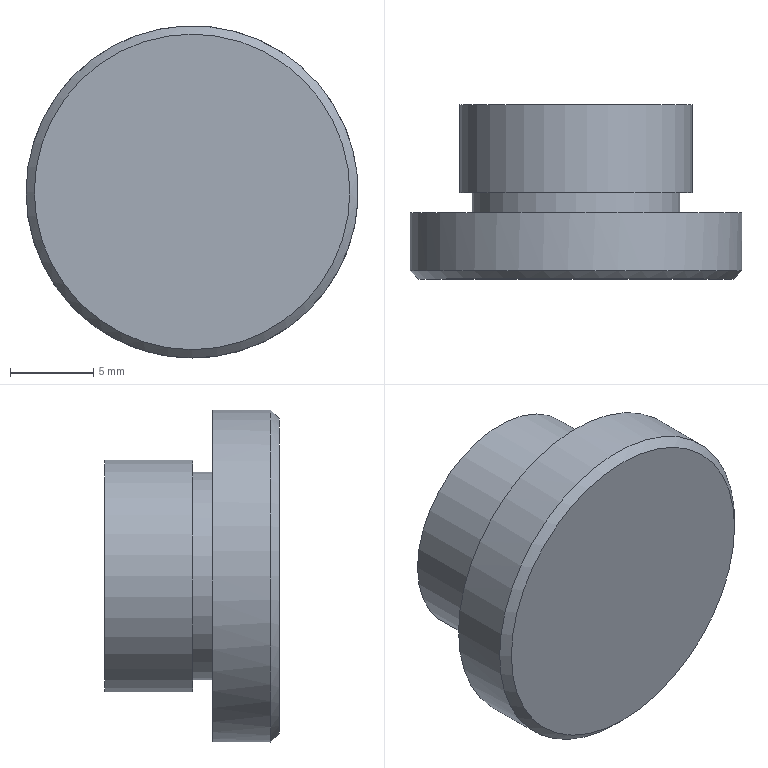Component | NX | END_CAP | 1 solid | 10 faces | box 20 x 10.5 x 20 mm | volume 1936 mm3 | plane 5 | cylinder 4 | cone 1 | commonest cylinder face diameters 20 x1 12.5 x1 14 x1 8 x1
STEP:
#1=CARTESIAN_POINT('',(0.,0.,0.));
#2=DIRECTION('',(0.,0.,1.));
#3=DIRECTION('',(1.,0.,0.));
#4=AXIS2_PLACEMENT_3D('',#1,#2,#3);
#5=CARTESIAN_POINT('',(13.994,-130.116,-10.));
#6=VERTEX_POINT('',#5);
#7=CARTESIAN_POINT('',(3.994,-130.116,-0.));
#8=VERTEX_POINT('',#7);
#9=CARTESIAN_POINT('',(13.994,-130.116,-0.));
#10=DIRECTION('',(0.,1.,0.));
#11=DIRECTION('',(0.,0.,-1.));
#12=AXIS2_PLACEMENT_3D('',#9,#10,#11);
#13=CIRCLE('',#12,10.);
#14=CARTESIAN_POINT('',(13.994,-126.616,-0.));
#15=DIRECTION('',(0.,-1.,0.));
#16=DIRECTION('',(0.,0.,1.));
#17=AXIS2_PLACEMENT_3D('',#14,#15,#16);
#18=CYLINDRICAL_SURFACE('',#17,10.);
#19=CARTESIAN_POINT('',(3.142,3.5));
#20=DIRECTION('',(-1.,0.));
#21=VECTOR('',#20,1.);
#22=LINE('',#19,#21);
#23=(GEOMETRIC_REPRESENTATION_CONTEXT(2)PARAMETRIC_REPRESENTATION_CONTEXT()REPRESENTATION_CONTEXT('',''));
#24=DEFINITIONAL_REPRESENTATION('',(#22),#23);
#25=PCURVE('',#18,#24);
#26=CARTESIAN_POINT('',(13.994,-130.116,-0.));
#27=DIRECTION('',(0.,1.,0.));
#28=DIRECTION('',(0.,0.,-1.));
#29=AXIS2_PLACEMENT_3D('',#26,#27,#28);
#30=CONICAL_SURFACE('',#29,10.,0.7854);
#31=CARTESIAN_POINT('',(0.,0.));
#32=DIRECTION('',(1.,0.));
#33=VECTOR('',#32,1.);
#34=LINE('',#31,#33);
#35=(GEOMETRIC_REPRESENTATION_CONTEXT(2)PARAMETRIC_REPRESENTATION_CONTEXT()REPRESENTATION_CONTEXT('',''));
#36=DEFINITIONAL_REPRESENTATION('',(#34),#35);
#37=PCURVE('',#30,#36);
#38=SURFACE_CURVE('',#13,(#25,#37),.PCURVE_S1.);
#39=EDGE_CURVE('',#6,#8,#38,.T.);
#40=ORIENTED_EDGE('',*,*,#39,.T.);
#41=CARTESIAN_POINT('',(3.994,-126.616,-0.));
#42=VERTEX_POINT('',#41);
#43=CARTESIAN_POINT('',(3.994,-126.616,-0.));
#44=CARTESIAN_POINT('',(3.994,-130.116,-0.));
#45=B_SPLINE_CURVE_WITH_KNOTS('',1,(#43,#44),.UNSPECIFIED.,.F.,.F.,(2,2),(0.,3.5),.PIECEWISE_BEZIER_KNOTS.);
#46=CARTESIAN_POINT('',(1.571,0.));
#47=DIRECTION('',(0.,1.));
#48=VECTOR('',#47,1.);
#49=LINE('',#46,#48);
#50=(GEOMETRIC_REPRESENTATION_CONTEXT(2)PARAMETRIC_REPRESENTATION_CONTEXT()REPRESENTATION_CONTEXT('',''));
#51=DEFINITIONAL_REPRESENTATION('',(#49),#50);
#52=PCURVE('',#18,#51);
#53=CARTESIAN_POINT('',(7.854,0.));
#54=DIRECTION('',(0.,1.));
#55=VECTOR('',#54,1.);
#56=LINE('',#53,#55);
#57=(GEOMETRIC_REPRESENTATION_CONTEXT(2)PARAMETRIC_REPRESENTATION_CONTEXT()REPRESENTATION_CONTEXT('',''));
#58=DEFINITIONAL_REPRESENTATION('',(#56),#57);
#59=PCURVE('',#18,#58);
#60=SEAM_CURVE('',#45,(#52,#59),.PCURVE_S1.);
#61=EDGE_CURVE('',#42,#8,#60,.T.);
#62=ORIENTED_EDGE('',*,*,#61,.F.);
#63=CARTESIAN_POINT('',(13.994,-126.616,-0.));
#64=DIRECTION('',(0.,1.,0.));
#65=DIRECTION('',(-1.,0.,-0.));
#66=AXIS2_PLACEMENT_3D('',#63,#64,#65);
#67=CIRCLE('',#66,10.);
#68=CARTESIAN_POINT('',(7.854,0.));
#69=DIRECTION('',(-1.,0.));
#70=VECTOR('',#69,1.);
#71=LINE('',#68,#70);
#72=(GEOMETRIC_REPRESENTATION_CONTEXT(2)PARAMETRIC_REPRESENTATION_CONTEXT()REPRESENTATION_CONTEXT('',''));
#73=DEFINITIONAL_REPRESENTATION('',(#71),#72);
#74=PCURVE('',#18,#73);
#75=CARTESIAN_POINT('',(13.994,-126.616,-0.));
#76=DIRECTION('',(0.,1.,0.));
#77=DIRECTION('',(0.,0.,-1.));
#78=AXIS2_PLACEMENT_3D('',#75,#76,#77);
#79=PLANE('',#78);
#80=CARTESIAN_POINT('',(0.,0.));
#81=DIRECTION('',(0.,1.));
#82=AXIS2_PLACEMENT_2D('',#80,#81);
#83=CIRCLE('',#82,10.);
#84=(GEOMETRIC_REPRESENTATION_CONTEXT(2)PARAMETRIC_REPRESENTATION_CONTEXT()REPRESENTATION_CONTEXT('',''));
#85=DEFINITIONAL_REPRESENTATION('',(#83),#84);
#86=PCURVE('',#79,#85);
#87=SURFACE_CURVE('',#67,(#74,#86),.PCURVE_S1.);
#88=EDGE_CURVE('',#42,#42,#87,.T.);
#89=ORIENTED_EDGE('',*,*,#88,.F.);
#90=ORIENTED_EDGE('',*,*,#61,.T.);
#91=CARTESIAN_POINT('',(13.994,-130.116,-0.));
#92=DIRECTION('',(0.,1.,0.));
#93=DIRECTION('',(0.,0.,-1.));
#94=AXIS2_PLACEMENT_3D('',#91,#92,#93);
#95=CIRCLE('',#94,10.);
#96=CARTESIAN_POINT('',(9.425,3.5));
#97=DIRECTION('',(-1.,0.));
#98=VECTOR('',#97,1.);
#99=LINE('',#96,#98);
#100=(GEOMETRIC_REPRESENTATION_CONTEXT(2)PARAMETRIC_REPRESENTATION_CONTEXT()REPRESENTATION_CONTEXT('',''));
#101=DEFINITIONAL_REPRESENTATION('',(#99),#100);
#102=PCURVE('',#18,#101);
#103=CARTESIAN_POINT('',(0.,0.));
#104=DIRECTION('',(1.,0.));
#105=VECTOR('',#104,1.);
#106=LINE('',#103,#105);
#107=(GEOMETRIC_REPRESENTATION_CONTEXT(2)PARAMETRIC_REPRESENTATION_CONTEXT()REPRESENTATION_CONTEXT('',''));
#108=DEFINITIONAL_REPRESENTATION('',(#106),#107);
#109=PCURVE('',#30,#108);
#110=SURFACE_CURVE('',#95,(#102,#109),.PCURVE_S1.);
#111=EDGE_CURVE('',#8,#6,#110,.T.);
#112=ORIENTED_EDGE('',*,*,#111,.T.);
#113=EDGE_LOOP('',(#40,#62,#89,#90,#112));
#114=FACE_BOUND('',#113,.T.);
#115=ADVANCED_FACE('',(#114),#18,.T.);
#116=CARTESIAN_POINT('',(7.744,-126.616,-0.));
#117=VERTEX_POINT('',#116);
#118=CARTESIAN_POINT('',(13.994,-126.616,-0.));
#119=DIRECTION('',(0.,1.,0.));
#120=DIRECTION('',(-1.,0.,-0.));
#121=AXIS2_PLACEMENT_3D('',#118,#119,#120);
#122=CIRCLE('',#121,6.25);
#123=CARTESIAN_POINT('',(0.,0.));
#124=DIRECTION('',(0.,1.));
#125=AXIS2_PLACEMENT_2D('',#123,#124);
#126=CIRCLE('',#125,6.25);
#127=(GEOMETRIC_REPRESENTATION_CONTEXT(2)PARAMETRIC_REPRESENTATION_CONTEXT()REPRESENTATION_CONTEXT('',''));
#128=DEFINITIONAL_REPRESENTATION('',(#126),#127);
#129=PCURVE('',#79,#128);
#130=CARTESIAN_POINT('',(13.994,-125.416,-0.));
#131=DIRECTION('',(0.,-1.,0.));
#132=DIRECTION('',(0.,0.,1.));
#133=AXIS2_PLACEMENT_3D('',#130,#131,#132);
#134=CYLINDRICAL_SURFACE('',#133,6.25);
#135=CARTESIAN_POINT('',(7.854,1.2));
#136=DIRECTION('',(-1.,0.));
#137=VECTOR('',#136,1.);
#138=LINE('',#135,#137);
#139=(GEOMETRIC_REPRESENTATION_CONTEXT(2)PARAMETRIC_REPRESENTATION_CONTEXT()REPRESENTATION_CONTEXT('',''));
#140=DEFINITIONAL_REPRESENTATION('',(#138),#139);
#141=PCURVE('',#134,#140);
#142=SURFACE_CURVE('',#122,(#129,#141),.PCURVE_S1.);
#143=EDGE_CURVE('',#117,#117,#142,.T.);
#144=ORIENTED_EDGE('',*,*,#143,.F.);
#145=EDGE_LOOP('',(#144));
#146=FACE_BOUND('',#145,.T.);
#147=ORIENTED_EDGE('',*,*,#88,.T.);
#148=EDGE_LOOP('',(#147));
#149=FACE_BOUND('',#148,.T.);
#150=ADVANCED_FACE('',(#146,#149),#79,.T.);
#151=CARTESIAN_POINT('',(13.994,-130.616,-9.5));
#152=VERTEX_POINT('',#151);
#153=CARTESIAN_POINT('',(13.994,-130.616,-0.));
#154=DIRECTION('',(0.,-1.,0.));
#155=DIRECTION('',(0.,0.,-1.));
#156=AXIS2_PLACEMENT_3D('',#153,#154,#155);
#157=CIRCLE('',#156,9.5);
#158=CARTESIAN_POINT('',(13.994,-130.616,-0.));
#159=DIRECTION('',(0.,1.,0.));
#160=DIRECTION('',(0.,0.,-1.));
#161=AXIS2_PLACEMENT_3D('',#158,#159,#160);
#162=PLANE('',#161);
#163=CARTESIAN_POINT('',(9.5,0.));
#164=CARTESIAN_POINT('',(9.5,-16.454));
#165=CARTESIAN_POINT('',(-4.75,-8.227));
#166=CARTESIAN_POINT('',(-19.,-0.));
#167=CARTESIAN_POINT('',(-4.75,8.227));
#168=CARTESIAN_POINT('',(9.5,16.454));
#169=CARTESIAN_POINT('',(9.5,0.));
#170=(BOUNDED_CURVE()B_SPLINE_CURVE(2,(#163,#164,#165,#166,#167,#168,#169),.UNSPECIFIED.,.T.,.F.)B_SPLINE_CURVE_WITH_KNOTS((1,2,2,2,2,1),(-2.094,0.,2.094,4.189,6.283,8.378),.UNSPECIFIED.)CURVE()GEOMETRIC_REPRESENTATION_ITEM()RATIONAL_B_SPLINE_CURVE((1.,0.5,1.,0.5,1.,0.5,1.))REPRESENTATION_ITEM(''));
#171=(GEOMETRIC_REPRESENTATION_CONTEXT(2)PARAMETRIC_REPRESENTATION_CONTEXT()REPRESENTATION_CONTEXT('',''));
#172=DEFINITIONAL_REPRESENTATION('',(#170),#171);
#173=PCURVE('',#162,#172);
#174=CARTESIAN_POINT('',(6.283,-0.5));
#175=DIRECTION('',(-1.,0.));
#176=VECTOR('',#175,1.);
#177=LINE('',#174,#176);
#178=(GEOMETRIC_REPRESENTATION_CONTEXT(2)PARAMETRIC_REPRESENTATION_CONTEXT()REPRESENTATION_CONTEXT('',''));
#179=DEFINITIONAL_REPRESENTATION('',(#177),#178);
#180=PCURVE('',#30,#179);
#181=SURFACE_CURVE('',#157,(#173,#180),.PCURVE_S1.);
#182=EDGE_CURVE('',#152,#152,#181,.T.);
#183=ORIENTED_EDGE('',*,*,#182,.T.);
#184=EDGE_LOOP('',(#183));
#185=FACE_BOUND('',#184,.T.);
#186=ADVANCED_FACE('',(#185),#162,.F.);
#187=CARTESIAN_POINT('',(7.744,-125.416,-0.));
#188=VERTEX_POINT('',#187);
#189=CARTESIAN_POINT('',(13.994,-125.416,-0.));
#190=DIRECTION('',(0.,1.,0.));
#191=DIRECTION('',(-1.,0.,-0.));
#192=AXIS2_PLACEMENT_3D('',#189,#190,#191);
#193=CIRCLE('',#192,6.25);
#194=CARTESIAN_POINT('',(7.854,0.));
#195=DIRECTION('',(-1.,0.));
#196=VECTOR('',#195,1.);
#197=LINE('',#194,#196);
#198=(GEOMETRIC_REPRESENTATION_CONTEXT(2)PARAMETRIC_REPRESENTATION_CONTEXT()REPRESENTATION_CONTEXT('',''));
#199=DEFINITIONAL_REPRESENTATION('',(#197),#198);
#200=PCURVE('',#134,#199);
#201=CARTESIAN_POINT('',(13.994,-125.416,-0.));
#202=DIRECTION('',(0.,1.,0.));
#203=DIRECTION('',(0.,0.,-1.));
#204=AXIS2_PLACEMENT_3D('',#201,#202,#203);
#205=PLANE('',#204);
#206=CARTESIAN_POINT('',(0.,0.));
#207=DIRECTION('',(0.,1.));
#208=AXIS2_PLACEMENT_2D('',#206,#207);
#209=CIRCLE('',#208,6.25);
#210=(GEOMETRIC_REPRESENTATION_CONTEXT(2)PARAMETRIC_REPRESENTATION_CONTEXT()REPRESENTATION_CONTEXT('',''));
#211=DEFINITIONAL_REPRESENTATION('',(#209),#210);
#212=PCURVE('',#205,#211);
#213=SURFACE_CURVE('',#193,(#200,#212),.PCURVE_S1.);
#214=EDGE_CURVE('',#188,#188,#213,.T.);
#215=ORIENTED_EDGE('',*,*,#214,.F.);
#216=CARTESIAN_POINT('',(7.744,-125.416,-0.));
#217=CARTESIAN_POINT('',(7.744,-126.616,-0.));
#218=B_SPLINE_CURVE_WITH_KNOTS('',1,(#216,#217),.UNSPECIFIED.,.F.,.F.,(2,2),(0.,1.2),.PIECEWISE_BEZIER_KNOTS.);
#219=CARTESIAN_POINT('',(7.854,0.));
#220=DIRECTION('',(0.,1.));
#221=VECTOR('',#220,1.);
#222=LINE('',#219,#221);
#223=(GEOMETRIC_REPRESENTATION_CONTEXT(2)PARAMETRIC_REPRESENTATION_CONTEXT()REPRESENTATION_CONTEXT('',''));
#224=DEFINITIONAL_REPRESENTATION('',(#222),#223);
#225=PCURVE('',#134,#224);
#226=CARTESIAN_POINT('',(1.571,0.));
#227=DIRECTION('',(0.,1.));
#228=VECTOR('',#227,1.);
#229=LINE('',#226,#228);
#230=(GEOMETRIC_REPRESENTATION_CONTEXT(2)PARAMETRIC_REPRESENTATION_CONTEXT()REPRESENTATION_CONTEXT('',''));
#231=DEFINITIONAL_REPRESENTATION('',(#229),#230);
#232=PCURVE('',#134,#231);
#233=SEAM_CURVE('',#218,(#225,#232),.PCURVE_S1.);
#234=EDGE_CURVE('',#188,#117,#233,.T.);
#235=ORIENTED_EDGE('',*,*,#234,.T.);
#236=ORIENTED_EDGE('',*,*,#143,.T.);
#237=ORIENTED_EDGE('',*,*,#234,.F.);
#238=EDGE_LOOP('',(#215,#235,#236,#237));
#239=FACE_BOUND('',#238,.T.);
#240=ADVANCED_FACE('',(#239),#134,.T.);
#241=CARTESIAN_POINT('',(6.994,-120.116,-0.));
#242=VERTEX_POINT('',#241);
#243=CARTESIAN_POINT('',(13.994,-120.116,-0.));
#244=DIRECTION('',(0.,1.,0.));
#245=DIRECTION('',(-1.,0.,-0.));
#246=AXIS2_PLACEMENT_3D('',#243,#244,#245);
#247=CIRCLE('',#246,7.);
#248=CARTESIAN_POINT('',(13.994,-120.116,-0.));
#249=DIRECTION('',(0.,-1.,0.));
#250=DIRECTION('',(0.,0.,1.));
#251=AXIS2_PLACEMENT_3D('',#248,#249,#250);
#252=CYLINDRICAL_SURFACE('',#251,7.);
#253=CARTESIAN_POINT('',(7.854,0.));
#254=DIRECTION('',(-1.,0.));
#255=VECTOR('',#254,1.);
#256=LINE('',#253,#255);
#257=(GEOMETRIC_REPRESENTATION_CONTEXT(2)PARAMETRIC_REPRESENTATION_CONTEXT()REPRESENTATION_CONTEXT('',''));
#258=DEFINITIONAL_REPRESENTATION('',(#256),#257);
#259=PCURVE('',#252,#258);
#260=CARTESIAN_POINT('',(13.994,-120.116,-0.));
#261=DIRECTION('',(0.,1.,0.));
#262=DIRECTION('',(0.,0.,-1.));
#263=AXIS2_PLACEMENT_3D('',#260,#261,#262);
#264=PLANE('',#263);
#265=CARTESIAN_POINT('',(0.,0.));
#266=DIRECTION('',(0.,1.));
#267=AXIS2_PLACEMENT_2D('',#265,#266);
#268=CIRCLE('',#267,7.);
#269=(GEOMETRIC_REPRESENTATION_CONTEXT(2)PARAMETRIC_REPRESENTATION_CONTEXT()REPRESENTATION_CONTEXT('',''));
#270=DEFINITIONAL_REPRESENTATION('',(#268),#269);
#271=PCURVE('',#264,#270);
#272=SURFACE_CURVE('',#247,(#259,#271),.PCURVE_S1.);
#273=EDGE_CURVE('',#242,#242,#272,.T.);
#274=ORIENTED_EDGE('',*,*,#273,.F.);
#275=CARTESIAN_POINT('',(6.994,-125.416,-0.));
#276=VERTEX_POINT('',#275);
#277=CARTESIAN_POINT('',(6.994,-120.116,-0.));
#278=CARTESIAN_POINT('',(6.994,-125.416,-0.));
#279=B_SPLINE_CURVE_WITH_KNOTS('',1,(#277,#278),.UNSPECIFIED.,.F.,.F.,(2,2),(0.,5.3),.PIECEWISE_BEZIER_KNOTS.);
#280=CARTESIAN_POINT('',(7.854,0.));
#281=DIRECTION('',(0.,1.));
#282=VECTOR('',#281,1.);
#283=LINE('',#280,#282);
#284=(GEOMETRIC_REPRESENTATION_CONTEXT(2)PARAMETRIC_REPRESENTATION_CONTEXT()REPRESENTATION_CONTEXT('',''));
#285=DEFINITIONAL_REPRESENTATION('',(#283),#284);
#286=PCURVE('',#252,#285);
#287=CARTESIAN_POINT('',(1.571,0.));
#288=DIRECTION('',(0.,1.));
#289=VECTOR('',#288,1.);
#290=LINE('',#287,#289);
#291=(GEOMETRIC_REPRESENTATION_CONTEXT(2)PARAMETRIC_REPRESENTATION_CONTEXT()REPRESENTATION_CONTEXT('',''));
#292=DEFINITIONAL_REPRESENTATION('',(#290),#291);
#293=PCURVE('',#252,#292);
#294=SEAM_CURVE('',#279,(#286,#293),.PCURVE_S1.);
#295=EDGE_CURVE('',#242,#276,#294,.T.);
#296=ORIENTED_EDGE('',*,*,#295,.T.);
#297=CARTESIAN_POINT('',(13.994,-125.416,-0.));
#298=DIRECTION('',(0.,1.,0.));
#299=DIRECTION('',(-1.,0.,-0.));
#300=AXIS2_PLACEMENT_3D('',#297,#298,#299);
#301=CIRCLE('',#300,7.);
#302=CARTESIAN_POINT('',(7.854,5.3));
#303=DIRECTION('',(-1.,0.));
#304=VECTOR('',#303,1.);
#305=LINE('',#302,#304);
#306=(GEOMETRIC_REPRESENTATION_CONTEXT(2)PARAMETRIC_REPRESENTATION_CONTEXT()REPRESENTATION_CONTEXT('',''));
#307=DEFINITIONAL_REPRESENTATION('',(#305),#306);
#308=PCURVE('',#252,#307);
#309=CARTESIAN_POINT('',(0.,0.));
#310=DIRECTION('',(0.,1.));
#311=AXIS2_PLACEMENT_2D('',#309,#310);
#312=CIRCLE('',#311,7.);
#313=(GEOMETRIC_REPRESENTATION_CONTEXT(2)PARAMETRIC_REPRESENTATION_CONTEXT()REPRESENTATION_CONTEXT('',''));
#314=DEFINITIONAL_REPRESENTATION('',(#312),#313);
#315=PCURVE('',#205,#314);
#316=SURFACE_CURVE('',#301,(#308,#315),.PCURVE_S1.);
#317=EDGE_CURVE('',#276,#276,#316,.T.);
#318=ORIENTED_EDGE('',*,*,#317,.T.);
#319=ORIENTED_EDGE('',*,*,#295,.F.);
#320=EDGE_LOOP('',(#274,#296,#318,#319));
#321=FACE_BOUND('',#320,.T.);
#322=ADVANCED_FACE('',(#321),#252,.T.);
#323=CARTESIAN_POINT('',(9.994,-120.116,-0.));
#324=VERTEX_POINT('',#323);
#325=CARTESIAN_POINT('',(13.994,-120.116,-0.));
#326=DIRECTION('',(0.,1.,0.));
#327=DIRECTION('',(-1.,0.,-0.));
#328=AXIS2_PLACEMENT_3D('',#325,#326,#327);
#329=CIRCLE('',#328,4.);
#330=CARTESIAN_POINT('',(0.,0.));
#331=DIRECTION('',(0.,1.));
#332=AXIS2_PLACEMENT_2D('',#330,#331);
#333=CIRCLE('',#332,4.);
#334=(GEOMETRIC_REPRESENTATION_CONTEXT(2)PARAMETRIC_REPRESENTATION_CONTEXT()REPRESENTATION_CONTEXT('',''));
#335=DEFINITIONAL_REPRESENTATION('',(#333),#334);
#336=PCURVE('',#264,#335);
#337=CARTESIAN_POINT('',(13.994,-125.616,-0.));
#338=DIRECTION('',(0.,1.,0.));
#339=DIRECTION('',(0.,0.,-1.));
#340=AXIS2_PLACEMENT_3D('',#337,#338,#339);
#341=CYLINDRICAL_SURFACE('',#340,4.);
#342=CARTESIAN_POINT('',(1.571,5.5));
#343=DIRECTION('',(1.,0.));
#344=VECTOR('',#343,1.);
#345=LINE('',#342,#344);
#346=(GEOMETRIC_REPRESENTATION_CONTEXT(2)PARAMETRIC_REPRESENTATION_CONTEXT()REPRESENTATION_CONTEXT('',''));
#347=DEFINITIONAL_REPRESENTATION('',(#345),#346);
#348=PCURVE('',#341,#347);
#349=SURFACE_CURVE('',#329,(#336,#348),.PCURVE_S1.);
#350=EDGE_CURVE('',#324,#324,#349,.T.);
#351=ORIENTED_EDGE('',*,*,#350,.F.);
#352=EDGE_LOOP('',(#351));
#353=FACE_BOUND('',#352,.T.);
#354=ORIENTED_EDGE('',*,*,#273,.T.);
#355=EDGE_LOOP('',(#354));
#356=FACE_BOUND('',#355,.T.);
#357=ADVANCED_FACE('',(#353,#356),#264,.T.);
#358=ORIENTED_EDGE('',*,*,#214,.T.);
#359=EDGE_LOOP('',(#358));
#360=FACE_BOUND('',#359,.T.);
#361=ORIENTED_EDGE('',*,*,#317,.F.);
#362=EDGE_LOOP('',(#361));
#363=FACE_BOUND('',#362,.T.);
#364=ADVANCED_FACE('',(#360,#363),#205,.F.);
#365=CARTESIAN_POINT('',(9.994,-125.616,-0.));
#366=VERTEX_POINT('',#365);
#367=CARTESIAN_POINT('',(13.994,-125.616,-0.));
#368=DIRECTION('',(0.,-1.,0.));
#369=DIRECTION('',(-1.,0.,-0.));
#370=AXIS2_PLACEMENT_3D('',#367,#368,#369);
#371=CIRCLE('',#370,4.);
#372=CARTESIAN_POINT('',(7.854,0.));
#373=DIRECTION('',(-1.,0.));
#374=VECTOR('',#373,1.);
#375=LINE('',#372,#374);
#376=(GEOMETRIC_REPRESENTATION_CONTEXT(2)PARAMETRIC_REPRESENTATION_CONTEXT()REPRESENTATION_CONTEXT('',''));
#377=DEFINITIONAL_REPRESENTATION('',(#375),#376);
#378=PCURVE('',#341,#377);
#379=CARTESIAN_POINT('',(13.994,-125.616,-0.));
#380=DIRECTION('',(0.,1.,0.));
#381=DIRECTION('',(0.,0.,-1.));
#382=AXIS2_PLACEMENT_3D('',#379,#380,#381);
#383=PLANE('',#382);
#384=CARTESIAN_POINT('',(0.,4.));
#385=CARTESIAN_POINT('',(6.928,4.));
#386=CARTESIAN_POINT('',(3.464,-2.));
#387=CARTESIAN_POINT('',(0.,-8.));
#388=CARTESIAN_POINT('',(-3.464,-2.));
#389=CARTESIAN_POINT('',(-6.928,4.));
#390=CARTESIAN_POINT('',(0.,4.));
#391=(BOUNDED_CURVE()B_SPLINE_CURVE(2,(#384,#385,#386,#387,#388,#389,#390),.UNSPECIFIED.,.T.,.F.)B_SPLINE_CURVE_WITH_KNOTS((1,2,2,2,2,1),(-2.094,0.,2.094,4.189,6.283,8.378),.UNSPECIFIED.)CURVE()GEOMETRIC_REPRESENTATION_ITEM()RATIONAL_B_SPLINE_CURVE((1.,0.5,1.,0.5,1.,0.5,1.))REPRESENTATION_ITEM(''));
#392=(GEOMETRIC_REPRESENTATION_CONTEXT(2)PARAMETRIC_REPRESENTATION_CONTEXT()REPRESENTATION_CONTEXT('',''));
#393=DEFINITIONAL_REPRESENTATION('',(#391),#392);
#394=PCURVE('',#383,#393);
#395=SURFACE_CURVE('',#371,(#378,#394),.PCURVE_S1.);
#396=EDGE_CURVE('',#366,#366,#395,.T.);
#397=ORIENTED_EDGE('',*,*,#396,.F.);
#398=CARTESIAN_POINT('',(9.994,-125.616,-0.));
#399=CARTESIAN_POINT('',(9.994,-120.116,-0.));
#400=B_SPLINE_CURVE_WITH_KNOTS('',1,(#398,#399),.UNSPECIFIED.,.F.,.F.,(2,2),(0.,5.5),.PIECEWISE_BEZIER_KNOTS.);
#401=CARTESIAN_POINT('',(7.854,0.));
#402=DIRECTION('',(0.,1.));
#403=VECTOR('',#402,1.);
#404=LINE('',#401,#403);
#405=(GEOMETRIC_REPRESENTATION_CONTEXT(2)PARAMETRIC_REPRESENTATION_CONTEXT()REPRESENTATION_CONTEXT('',''));
#406=DEFINITIONAL_REPRESENTATION('',(#404),#405);
#407=PCURVE('',#341,#406);
#408=CARTESIAN_POINT('',(1.571,0.));
#409=DIRECTION('',(0.,1.));
#410=VECTOR('',#409,1.);
#411=LINE('',#408,#410);
#412=(GEOMETRIC_REPRESENTATION_CONTEXT(2)PARAMETRIC_REPRESENTATION_CONTEXT()REPRESENTATION_CONTEXT('',''));
#413=DEFINITIONAL_REPRESENTATION('',(#411),#412);
#414=PCURVE('',#341,#413);
#415=SEAM_CURVE('',#400,(#407,#414),.PCURVE_S1.);
#416=EDGE_CURVE('',#366,#324,#415,.T.);
#417=ORIENTED_EDGE('',*,*,#416,.T.);
#418=ORIENTED_EDGE('',*,*,#350,.F.);
#419=ORIENTED_EDGE('',*,*,#416,.F.);
#420=EDGE_LOOP('',(#397,#417,#418,#419));
#421=FACE_BOUND('',#420,.F.);
#422=ADVANCED_FACE('',(#421),#341,.F.);
#423=ORIENTED_EDGE('',*,*,#396,.F.);
#424=EDGE_LOOP('',(#423));
#425=FACE_BOUND('',#424,.T.);
#426=ADVANCED_FACE('',(#425),#383,.T.);
#427=ORIENTED_EDGE('',*,*,#182,.F.);
#428=CARTESIAN_POINT('',(13.994,-130.616,-9.5));
#429=CARTESIAN_POINT('',(13.994,-130.116,-10.));
#430=B_SPLINE_CURVE_WITH_KNOTS('',1,(#428,#429),.UNSPECIFIED.,.F.,.F.,(2,2),(-0.7071,0.),.PIECEWISE_BEZIER_KNOTS.);
#431=CARTESIAN_POINT('',(6.283,0.));
#432=DIRECTION('',(0.,1.));
#433=VECTOR('',#432,1.);
#434=LINE('',#431,#433);
#435=(GEOMETRIC_REPRESENTATION_CONTEXT(2)PARAMETRIC_REPRESENTATION_CONTEXT()REPRESENTATION_CONTEXT('',''));
#436=DEFINITIONAL_REPRESENTATION('',(#434),#435);
#437=PCURVE('',#30,#436);
#438=CARTESIAN_POINT('',(0.,0.));
#439=DIRECTION('',(0.,1.));
#440=VECTOR('',#439,1.);
#441=LINE('',#438,#440);
#442=(GEOMETRIC_REPRESENTATION_CONTEXT(2)PARAMETRIC_REPRESENTATION_CONTEXT()REPRESENTATION_CONTEXT('',''));
#443=DEFINITIONAL_REPRESENTATION('',(#441),#442);
#444=PCURVE('',#30,#443);
#445=SEAM_CURVE('',#430,(#437,#444),.PCURVE_S1.);
#446=EDGE_CURVE('',#152,#6,#445,.T.);
#447=ORIENTED_EDGE('',*,*,#446,.T.);
#448=ORIENTED_EDGE('',*,*,#111,.F.);
#449=ORIENTED_EDGE('',*,*,#39,.F.);
#450=ORIENTED_EDGE('',*,*,#446,.F.);
#451=EDGE_LOOP('',(#427,#447,#448,#449,#450));
#452=FACE_BOUND('',#451,.T.);
#453=ADVANCED_FACE('',(#452),#30,.T.);
#454=CLOSED_SHELL('',(#115,#150,#186,#240,#322,#357,#364,#422,#426,#453));
#455=MANIFOLD_SOLID_BREP('',#454);
#456=(LENGTH_UNIT()NAMED_UNIT(*)SI_UNIT(.MILLI.,.METRE.));
#457=UNCERTAINTY_MEASURE_WITH_UNIT(LENGTH_MEASURE(0.00001),#456,'','');
#458=(NAMED_UNIT(*)PLANE_ANGLE_UNIT()SI_UNIT($,.RADIAN.));
#459=(NAMED_UNIT(*)SI_UNIT($,.STERADIAN.)SOLID_ANGLE_UNIT());
#460=(GEOMETRIC_REPRESENTATION_CONTEXT(3)GLOBAL_UNCERTAINTY_ASSIGNED_CONTEXT((#457))GLOBAL_UNIT_ASSIGNED_CONTEXT((#456,#458,#459))REPRESENTATION_CONTEXT('',''));
#461=ADVANCED_BREP_SHAPE_REPRESENTATION('',(#4,#455),#460);